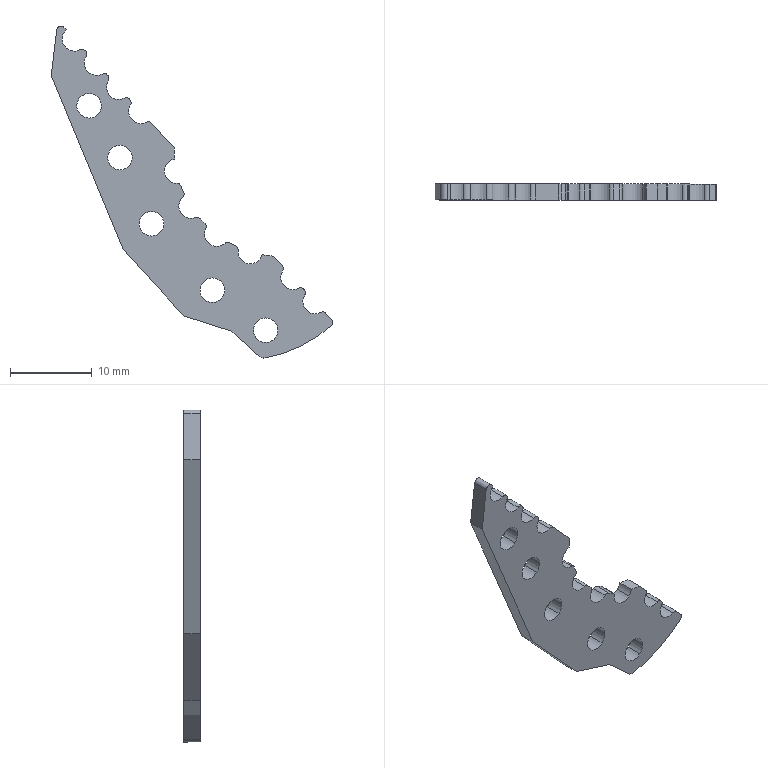Component | SolidWorks | PartNew2-1 | 1 solid | 57 faces | volume 724 mm3 | cylinder 42 | plane 12 | spline 3 | commonest cylinder face diameters 3 x21 1 x14 26.643 x5 2 x1 33.55 x1